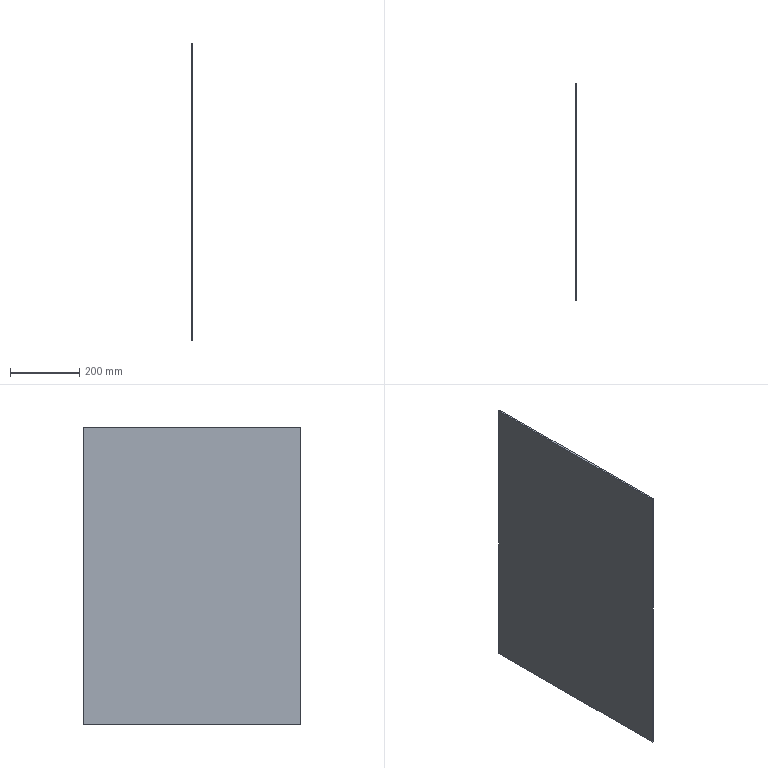Component | SolidWorks | 858X628X5-2 | 1 solid | 6 faces | box 5 x 628 x 858 mm | volume 2694120 mm3 | plane 6
build123d program:
from build123d import *

# Parameters (mm, degrees)
SKETCH1_W           = 858
SKETCH1_H           = 628
BOSS_EXTRUDE1_DEPTH = 5


with BuildPart() as part:
    # Sketch1 → Boss-Extrude1 (new body)
    with BuildSketch(Plane.XY):
        with Locations((429, -314)):
            Rectangle(SKETCH1_W, SKETCH1_H)
    extrude(amount=BOSS_EXTRUDE1_DEPTH)


solid = part.part

# Placed as in the assembly
solid = solid.moved(Location((-17.047, 631.523, 429), (0, 90, 0)))
STEP:
#1=CARTESIAN_POINT('',(-0.4743,24.863,-16.89));
#2=VERTEX_POINT('',#1);
#3=CARTESIAN_POINT('',(-0.4743,0.1387,-16.89));
#4=VERTEX_POINT('',#3);
#5=CARTESIAN_POINT('',(-0.4743,24.863,-16.89));
#6=DIRECTION('',(-0.,-1.,-0.));
#7=VECTOR('',#6,39.37);
#8=LINE('',#5,#7);
#9=EDGE_CURVE('',#2,#4,#8,.T.);
#10=ORIENTED_EDGE('',*,*,#9,.T.);
#11=CARTESIAN_POINT('',(-0.6711,0.1387,-16.89));
#12=VERTEX_POINT('',#11);
#13=CARTESIAN_POINT('',(-0.6711,0.1387,-16.89));
#14=DIRECTION('',(1.,-0.,0.));
#15=VECTOR('',#14,39.37);
#16=LINE('',#13,#15);
#17=EDGE_CURVE('',#12,#4,#16,.T.);
#18=ORIENTED_EDGE('',*,*,#17,.F.);
#19=CARTESIAN_POINT('',(-0.6711,24.863,-16.89));
#20=VERTEX_POINT('',#19);
#21=CARTESIAN_POINT('',(-0.6711,24.863,-16.89));
#22=DIRECTION('',(-0.,-1.,-0.));
#23=VECTOR('',#22,39.37);
#24=LINE('',#21,#23);
#25=EDGE_CURVE('',#20,#12,#24,.T.);
#26=ORIENTED_EDGE('',*,*,#25,.F.);
#27=CARTESIAN_POINT('',(-0.6711,24.863,-16.89));
#28=DIRECTION('',(1.,-0.,0.));
#29=VECTOR('',#28,39.37);
#30=LINE('',#27,#29);
#31=EDGE_CURVE('',#20,#2,#30,.T.);
#32=ORIENTED_EDGE('',*,*,#31,.T.);
#33=EDGE_LOOP('',(#10,#18,#26,#32));
#34=FACE_OUTER_BOUND('',#33,.T.);
#35=CARTESIAN_POINT('',(-0.6711,24.863,-16.89));
#36=DIRECTION('',(-0.,-0.,1.));
#37=DIRECTION('',(0.,1.,0.));
#38=AXIS2_PLACEMENT_3D('',#35,#36,#37);
#39=PLANE('',#38);
#40=ADVANCED_FACE('',(#34),#39,.F.);
#41=CARTESIAN_POINT('',(-0.4743,0.1387,16.89));
#42=VERTEX_POINT('',#41);
#43=CARTESIAN_POINT('',(-0.4743,0.1387,-16.89));
#44=DIRECTION('',(-0.,-0.,1.));
#45=VECTOR('',#44,39.37);
#46=LINE('',#43,#45);
#47=EDGE_CURVE('',#4,#42,#46,.T.);
#48=ORIENTED_EDGE('',*,*,#47,.T.);
#49=CARTESIAN_POINT('',(-0.6711,0.1387,16.89));
#50=VERTEX_POINT('',#49);
#51=CARTESIAN_POINT('',(-0.6711,0.1387,16.89));
#52=DIRECTION('',(1.,-0.,0.));
#53=VECTOR('',#52,39.37);
#54=LINE('',#51,#53);
#55=EDGE_CURVE('',#50,#42,#54,.T.);
#56=ORIENTED_EDGE('',*,*,#55,.F.);
#57=CARTESIAN_POINT('',(-0.6711,0.1387,-16.89));
#58=DIRECTION('',(-0.,-0.,1.));
#59=VECTOR('',#58,39.37);
#60=LINE('',#57,#59);
#61=EDGE_CURVE('',#12,#50,#60,.T.);
#62=ORIENTED_EDGE('',*,*,#61,.F.);
#63=ORIENTED_EDGE('',*,*,#17,.T.);
#64=EDGE_LOOP('',(#48,#56,#62,#63));
#65=FACE_OUTER_BOUND('',#64,.T.);
#66=CARTESIAN_POINT('',(-0.6711,0.1387,-16.89));
#67=DIRECTION('',(0.,1.,0.));
#68=DIRECTION('',(-1.,0.,-0.));
#69=AXIS2_PLACEMENT_3D('',#66,#67,#68);
#70=PLANE('',#69);
#71=ADVANCED_FACE('',(#65),#70,.F.);
#72=CARTESIAN_POINT('',(-0.4743,24.863,16.89));
#73=VERTEX_POINT('',#72);
#74=CARTESIAN_POINT('',(-0.4743,24.863,16.89));
#75=DIRECTION('',(0.,1.,0.));
#76=VECTOR('',#75,39.37);
#77=LINE('',#74,#76);
#78=EDGE_CURVE('',#42,#73,#77,.T.);
#79=ORIENTED_EDGE('',*,*,#78,.T.);
#80=CARTESIAN_POINT('',(-0.6711,24.863,16.89));
#81=VERTEX_POINT('',#80);
#82=CARTESIAN_POINT('',(-0.6711,24.863,16.89));
#83=DIRECTION('',(1.,-0.,0.));
#84=VECTOR('',#83,39.37);
#85=LINE('',#82,#84);
#86=EDGE_CURVE('',#81,#73,#85,.T.);
#87=ORIENTED_EDGE('',*,*,#86,.F.);
#88=CARTESIAN_POINT('',(-0.6711,24.863,16.89));
#89=DIRECTION('',(0.,1.,0.));
#90=VECTOR('',#89,39.37);
#91=LINE('',#88,#90);
#92=EDGE_CURVE('',#50,#81,#91,.T.);
#93=ORIENTED_EDGE('',*,*,#92,.F.);
#94=ORIENTED_EDGE('',*,*,#55,.T.);
#95=EDGE_LOOP('',(#79,#87,#93,#94));
#96=FACE_OUTER_BOUND('',#95,.T.);
#97=CARTESIAN_POINT('',(-0.6711,24.863,16.89));
#98=DIRECTION('',(0.,0.,-1.));
#99=DIRECTION('',(-0.,-1.,-0.));
#100=AXIS2_PLACEMENT_3D('',#97,#98,#99);
#101=PLANE('',#100);
#102=ADVANCED_FACE('',(#96),#101,.F.);
#103=CARTESIAN_POINT('',(-0.4743,24.863,-16.89));
#104=DIRECTION('',(0.,0.,-1.));
#105=VECTOR('',#104,39.37);
#106=LINE('',#103,#105);
#107=EDGE_CURVE('',#73,#2,#106,.T.);
#108=ORIENTED_EDGE('',*,*,#107,.T.);
#109=ORIENTED_EDGE('',*,*,#31,.F.);
#110=CARTESIAN_POINT('',(-0.6711,24.863,-16.89));
#111=DIRECTION('',(0.,0.,-1.));
#112=VECTOR('',#111,39.37);
#113=LINE('',#110,#112);
#114=EDGE_CURVE('',#81,#20,#113,.T.);
#115=ORIENTED_EDGE('',*,*,#114,.F.);
#116=ORIENTED_EDGE('',*,*,#86,.T.);
#117=EDGE_LOOP('',(#108,#109,#115,#116));
#118=FACE_OUTER_BOUND('',#117,.T.);
#119=CARTESIAN_POINT('',(-0.6711,24.863,-16.89));
#120=DIRECTION('',(-0.,-1.,-0.));
#121=DIRECTION('',(1.,-0.,0.));
#122=AXIS2_PLACEMENT_3D('',#119,#120,#121);
#123=PLANE('',#122);
#124=ADVANCED_FACE('',(#118),#123,.F.);
#125=ORIENTED_EDGE('',*,*,#25,.T.);
#126=ORIENTED_EDGE('',*,*,#61,.T.);
#127=ORIENTED_EDGE('',*,*,#92,.T.);
#128=ORIENTED_EDGE('',*,*,#114,.T.);
#129=EDGE_LOOP('',(#125,#126,#127,#128));
#130=FACE_OUTER_BOUND('',#129,.T.);
#131=CARTESIAN_POINT('',(-0.6711,24.863,-16.89));
#132=DIRECTION('',(-1.,0.,-0.));
#133=DIRECTION('',(-0.,-0.,1.));
#134=AXIS2_PLACEMENT_3D('',#131,#132,#133);
#135=PLANE('',#134);
#136=ADVANCED_FACE('',(#130),#135,.T.);
#137=ORIENTED_EDGE('',*,*,#9,.F.);
#138=ORIENTED_EDGE('',*,*,#107,.F.);
#139=ORIENTED_EDGE('',*,*,#78,.F.);
#140=ORIENTED_EDGE('',*,*,#47,.F.);
#141=EDGE_LOOP('',(#137,#138,#139,#140));
#142=FACE_OUTER_BOUND('',#141,.T.);
#143=CARTESIAN_POINT('',(-0.4743,24.863,-16.89));
#144=DIRECTION('',(-1.,0.,-0.));
#145=DIRECTION('',(-0.,-0.,1.));
#146=AXIS2_PLACEMENT_3D('',#143,#144,#145);
#147=PLANE('',#146);
#148=ADVANCED_FACE('',(#142),#147,.F.);
#149=CLOSED_SHELL('',(#40,#71,#102,#124,#136,#148));
#150=MANIFOLD_SOLID_BREP('',#149);
#151=CARTESIAN_POINT('',(0.,0.,0.));
#152=DIRECTION('',(0.,0.,1.));
#153=DIRECTION('',(1.,0.,0.));
#154=AXIS2_PLACEMENT_3D('',#151,#152,#153);
#155=(LENGTH_UNIT()NAMED_UNIT(*)SI_UNIT($,.METRE.));
#156=LENGTH_MEASURE_WITH_UNIT(LENGTH_MEASURE(0.0254),#155);
#157=DIMENSIONAL_EXPONENTS(1.,0.,0.,0.,0.,0.,0.);
#158=(CONVERSION_BASED_UNIT('',#156)LENGTH_UNIT()NAMED_UNIT(#157));
#159=UNCERTAINTY_MEASURE_WITH_UNIT(LENGTH_MEASURE(0.00001),#158,'','');
#160=(NAMED_UNIT(*)PLANE_ANGLE_UNIT()SI_UNIT($,.RADIAN.));
#161=(NAMED_UNIT(*)SI_UNIT($,.STERADIAN.)SOLID_ANGLE_UNIT());
#162=(GEOMETRIC_REPRESENTATION_CONTEXT(3)GLOBAL_UNCERTAINTY_ASSIGNED_CONTEXT((#159))GLOBAL_UNIT_ASSIGNED_CONTEXT((#158,#160,#161))REPRESENTATION_CONTEXT('',''));
#163=ADVANCED_BREP_SHAPE_REPRESENTATION('',(#150,#154),#162);
#164=COLOUR_RGB('',0.7922,0.8196,0.9333);
#165=FILL_AREA_STYLE_COLOUR('',#164);
#166=FILL_AREA_STYLE('',(#165));
#167=SURFACE_STYLE_FILL_AREA(#166);
#168=SURFACE_SIDE_STYLE('',(#167));
#169=SURFACE_STYLE_USAGE(.BOTH.,#168);
#170=PRESENTATION_STYLE_ASSIGNMENT((#169));
#171=STYLED_ITEM('',(#170),#150);
#172=PRESENTATION_LAYER_ASSIGNMENT('','',(#171));
#173=(LENGTH_UNIT()NAMED_UNIT(*)SI_UNIT($,.METRE.));
#174=LENGTH_MEASURE_WITH_UNIT(LENGTH_MEASURE(0.0254),#173);
#175=DIMENSIONAL_EXPONENTS(1.,0.,0.,0.,0.,0.,0.);
#176=(CONVERSION_BASED_UNIT('',#174)LENGTH_UNIT()NAMED_UNIT(#175));
#177=UNCERTAINTY_MEASURE_WITH_UNIT(LENGTH_MEASURE(0.00001),#176,'','');
#178=(NAMED_UNIT(*)PLANE_ANGLE_UNIT()SI_UNIT($,.RADIAN.));
#179=(NAMED_UNIT(*)SI_UNIT($,.STERADIAN.)SOLID_ANGLE_UNIT());
#180=(GEOMETRIC_REPRESENTATION_CONTEXT(3)GLOBAL_UNCERTAINTY_ASSIGNED_CONTEXT((#177))GLOBAL_UNIT_ASSIGNED_CONTEXT((#176,#178,#179))REPRESENTATION_CONTEXT('',''));
#181=MECHANICAL_DESIGN_GEOMETRIC_PRESENTATION_REPRESENTATION('',(#171),#180);